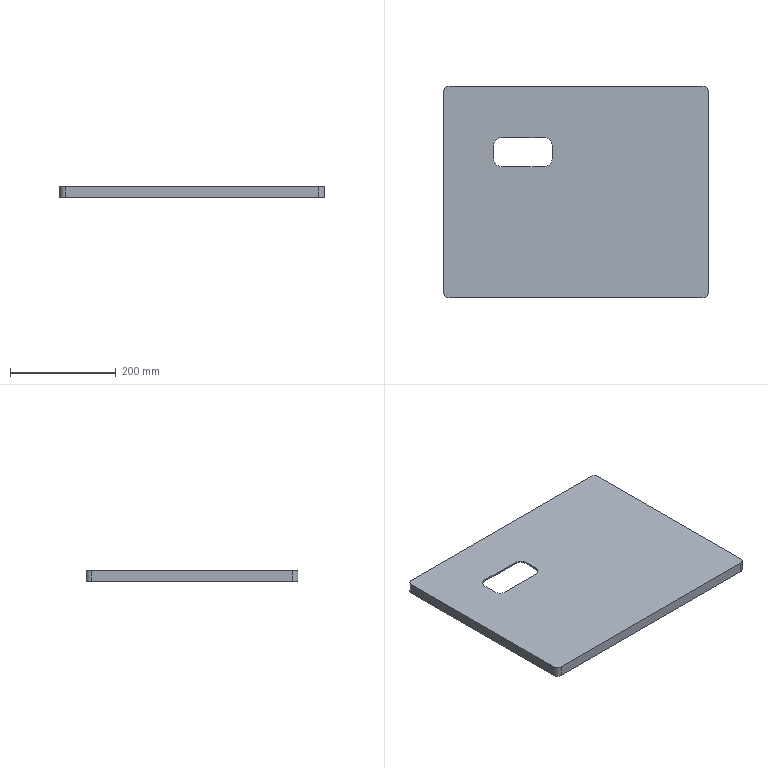Component | SolidWorks | LX-TSJ-16-1 | 1 solid | 27 faces | box 500 x 400 x 20 mm | volume 672509 mm3 | plane 15 | cylinder 12 | commonest cylinder face diameters 20 x4 14 x4 30 x4
STEP:
#1=COLOUR_RGB('',0.7922,0.8196,0.9333);
#2=FILL_AREA_STYLE_COLOUR('',#1);
#3=FILL_AREA_STYLE('',(#2));
#4=SURFACE_STYLE_FILL_AREA(#3);
#5=SURFACE_SIDE_STYLE('',(#4));
#6=SURFACE_STYLE_USAGE(.BOTH.,#5);
#7=PRESENTATION_STYLE_ASSIGNMENT((#6));
#8=CARTESIAN_POINT('',(-7.413,-19.336,-5.681));
#9=VERTEX_POINT('',#8);
#10=CARTESIAN_POINT('',(-7.413,-20.326,-5.681));
#11=VERTEX_POINT('',#10);
#12=CARTESIAN_POINT('',(-7.413,-30.275,-5.681));
#13=DIRECTION('',(0.,-1.,-0.));
#14=VECTOR('',#13,39.37);
#15=LINE('',#12,#14);
#16=EDGE_CURVE('',#9,#11,#15,.T.);
#17=ORIENTED_EDGE('',*,*,#16,.T.);
#18=CARTESIAN_POINT('',(-8.004,-20.917,-5.681));
#19=VERTEX_POINT('',#18);
#20=CARTESIAN_POINT('',(-8.004,-20.326,-5.681));
#21=DIRECTION('',(0.,0.,-1.));
#22=DIRECTION('',(-1.,0.,0.));
#23=AXIS2_PLACEMENT_3D('',#20,#21,#22);
#24=CIRCLE('',#23,0.5906);
#25=EDGE_CURVE('',#11,#19,#24,.T.);
#26=ORIENTED_EDGE('',*,*,#25,.T.);
#27=CARTESIAN_POINT('',(-11.166,-20.917,-5.681));
#28=VERTEX_POINT('',#27);
#29=CARTESIAN_POINT('',(3.818,-20.917,-5.681));
#30=DIRECTION('',(-1.,-0.,-0.));
#31=VECTOR('',#30,39.37);
#32=LINE('',#29,#31);
#33=EDGE_CURVE('',#19,#28,#32,.T.);
#34=ORIENTED_EDGE('',*,*,#33,.T.);
#35=CARTESIAN_POINT('',(-11.756,-20.326,-5.681));
#36=VERTEX_POINT('',#35);
#37=CARTESIAN_POINT('',(-11.166,-20.326,-5.681));
#38=DIRECTION('',(0.,0.,-1.));
#39=DIRECTION('',(-1.,0.,0.));
#40=AXIS2_PLACEMENT_3D('',#37,#38,#39);
#41=CIRCLE('',#40,0.5906);
#42=EDGE_CURVE('',#28,#36,#41,.T.);
#43=ORIENTED_EDGE('',*,*,#42,.T.);
#44=CARTESIAN_POINT('',(-11.756,-19.336,-5.681));
#45=VERTEX_POINT('',#44);
#46=CARTESIAN_POINT('',(-11.756,-30.275,-5.681));
#47=DIRECTION('',(-0.,1.,0.));
#48=VECTOR('',#47,39.37);
#49=LINE('',#46,#48);
#50=EDGE_CURVE('',#36,#45,#49,.T.);
#51=ORIENTED_EDGE('',*,*,#50,.T.);
#52=CARTESIAN_POINT('',(-11.166,-18.745,-5.681));
#53=VERTEX_POINT('',#52);
#54=CARTESIAN_POINT('',(-11.166,-19.336,-5.681));
#55=DIRECTION('',(0.,0.,-1.));
#56=DIRECTION('',(-1.,0.,0.));
#57=AXIS2_PLACEMENT_3D('',#54,#55,#56);
#58=CIRCLE('',#57,0.5906);
#59=EDGE_CURVE('',#45,#53,#58,.T.);
#60=ORIENTED_EDGE('',*,*,#59,.T.);
#61=CARTESIAN_POINT('',(-8.004,-18.745,-5.681));
#62=VERTEX_POINT('',#61);
#63=CARTESIAN_POINT('',(3.818,-18.745,-5.681));
#64=DIRECTION('',(1.,0.,0.));
#65=VECTOR('',#64,39.37);
#66=LINE('',#63,#65);
#67=EDGE_CURVE('',#53,#62,#66,.T.);
#68=ORIENTED_EDGE('',*,*,#67,.T.);
#69=CARTESIAN_POINT('',(-8.004,-19.336,-5.681));
#70=DIRECTION('',(0.,0.,-1.));
#71=DIRECTION('',(-1.,0.,0.));
#72=AXIS2_PLACEMENT_3D('',#69,#70,#71);
#73=CIRCLE('',#72,0.5906);
#74=EDGE_CURVE('',#62,#9,#73,.T.);
#75=ORIENTED_EDGE('',*,*,#74,.T.);
#76=EDGE_LOOP('',(#17,#26,#34,#43,#51,#60,#68,#75));
#77=FACE_BOUND('',#76,.T.);
#78=CARTESIAN_POINT('',(4.212,-15.314,-5.681));
#79=VERTEX_POINT('',#78);
#80=CARTESIAN_POINT('',(4.212,-30.275,-5.681));
#81=VERTEX_POINT('',#80);
#82=CARTESIAN_POINT('',(4.212,-30.275,-5.681));
#83=DIRECTION('',(0.,-1.,-0.));
#84=VECTOR('',#83,39.37);
#85=LINE('',#82,#84);
#86=EDGE_CURVE('',#79,#81,#85,.T.);
#87=ORIENTED_EDGE('',*,*,#86,.F.);
#88=CARTESIAN_POINT('',(3.818,-14.92,-5.681));
#89=VERTEX_POINT('',#88);
#90=CARTESIAN_POINT('',(3.818,-15.314,-5.681));
#91=DIRECTION('',(0.,0.,-1.));
#92=DIRECTION('',(1.,0.,0.));
#93=AXIS2_PLACEMENT_3D('',#90,#91,#92);
#94=CIRCLE('',#93,0.3937);
#95=EDGE_CURVE('',#89,#79,#94,.T.);
#96=ORIENTED_EDGE('',*,*,#95,.F.);
#97=CARTESIAN_POINT('',(-15.08,-14.92,-5.681));
#98=VERTEX_POINT('',#97);
#99=CARTESIAN_POINT('',(3.818,-14.92,-5.681));
#100=DIRECTION('',(1.,0.,0.));
#101=VECTOR('',#100,39.37);
#102=LINE('',#99,#101);
#103=EDGE_CURVE('',#98,#89,#102,.T.);
#104=ORIENTED_EDGE('',*,*,#103,.F.);
#105=CARTESIAN_POINT('',(-15.473,-15.314,-5.681));
#106=VERTEX_POINT('',#105);
#107=CARTESIAN_POINT('',(-15.08,-15.314,-5.681));
#108=DIRECTION('',(0.,0.,-1.));
#109=DIRECTION('',(1.,0.,0.));
#110=AXIS2_PLACEMENT_3D('',#107,#108,#109);
#111=CIRCLE('',#110,0.3937);
#112=EDGE_CURVE('',#106,#98,#111,.T.);
#113=ORIENTED_EDGE('',*,*,#112,.F.);
#114=CARTESIAN_POINT('',(-15.473,-30.275,-5.681));
#115=VERTEX_POINT('',#114);
#116=CARTESIAN_POINT('',(-15.473,-30.275,-5.681));
#117=DIRECTION('',(-0.,1.,0.));
#118=VECTOR('',#117,39.37);
#119=LINE('',#116,#118);
#120=EDGE_CURVE('',#115,#106,#119,.T.);
#121=ORIENTED_EDGE('',*,*,#120,.F.);
#122=CARTESIAN_POINT('',(-15.08,-30.668,-5.681));
#123=VERTEX_POINT('',#122);
#124=CARTESIAN_POINT('',(-15.08,-30.275,-5.681));
#125=DIRECTION('',(0.,0.,-1.));
#126=DIRECTION('',(1.,0.,0.));
#127=AXIS2_PLACEMENT_3D('',#124,#125,#126);
#128=CIRCLE('',#127,0.3937);
#129=EDGE_CURVE('',#123,#115,#128,.T.);
#130=ORIENTED_EDGE('',*,*,#129,.F.);
#131=CARTESIAN_POINT('',(3.818,-30.668,-5.681));
#132=VERTEX_POINT('',#131);
#133=CARTESIAN_POINT('',(3.818,-30.668,-5.681));
#134=DIRECTION('',(-1.,-0.,-0.));
#135=VECTOR('',#134,39.37);
#136=LINE('',#133,#135);
#137=EDGE_CURVE('',#132,#123,#136,.T.);
#138=ORIENTED_EDGE('',*,*,#137,.F.);
#139=CARTESIAN_POINT('',(3.818,-30.275,-5.681));
#140=DIRECTION('',(0.,0.,-1.));
#141=DIRECTION('',(1.,0.,0.));
#142=AXIS2_PLACEMENT_3D('',#139,#140,#141);
#143=CIRCLE('',#142,0.3937);
#144=EDGE_CURVE('',#81,#132,#143,.T.);
#145=ORIENTED_EDGE('',*,*,#144,.F.);
#146=EDGE_LOOP('',(#87,#96,#104,#113,#121,#130,#138,#145));
#147=FACE_OUTER_BOUND('',#146,.T.);
#148=CARTESIAN_POINT('',(3.818,-30.275,-5.681));
#149=DIRECTION('',(0.,0.,-1.));
#150=DIRECTION('',(-1.,-0.,-0.));
#151=AXIS2_PLACEMENT_3D('',#148,#149,#150);
#152=PLANE('',#151);
#153=ADVANCED_FACE('',(#77,#147),#152,.F.);
#154=CARTESIAN_POINT('',(3.818,-30.668,-6.468));
#155=VERTEX_POINT('',#154);
#156=CARTESIAN_POINT('',(4.212,-30.275,-6.468));
#157=VERTEX_POINT('',#156);
#158=CARTESIAN_POINT('',(3.818,-30.275,-6.468));
#159=DIRECTION('',(-0.,-0.,1.));
#160=DIRECTION('',(1.,0.,0.));
#161=AXIS2_PLACEMENT_3D('',#158,#159,#160);
#162=CIRCLE('',#161,0.3937);
#163=EDGE_CURVE('',#155,#157,#162,.T.);
#164=ORIENTED_EDGE('',*,*,#163,.T.);
#165=CARTESIAN_POINT('',(4.212,-30.275,-6.468));
#166=DIRECTION('',(-0.,-0.,1.));
#167=VECTOR('',#166,39.37);
#168=LINE('',#165,#167);
#169=EDGE_CURVE('',#157,#81,#168,.T.);
#170=ORIENTED_EDGE('',*,*,#169,.T.);
#171=ORIENTED_EDGE('',*,*,#144,.T.);
#172=CARTESIAN_POINT('',(3.818,-30.668,-6.468));
#173=DIRECTION('',(0.,0.,-1.));
#174=VECTOR('',#173,39.37);
#175=LINE('',#172,#174);
#176=EDGE_CURVE('',#132,#155,#175,.T.);
#177=ORIENTED_EDGE('',*,*,#176,.T.);
#178=EDGE_LOOP('',(#164,#170,#171,#177));
#179=FACE_OUTER_BOUND('',#178,.T.);
#180=CARTESIAN_POINT('',(3.818,-30.275,-6.468));
#181=DIRECTION('',(-0.,-0.,1.));
#182=DIRECTION('',(1.,0.,0.));
#183=AXIS2_PLACEMENT_3D('',#180,#181,#182);
#184=CYLINDRICAL_SURFACE('',#183,0.3937);
#185=ADVANCED_FACE('',(#179),#184,.T.);
#186=ORIENTED_EDGE('',*,*,#169,.F.);
#187=CARTESIAN_POINT('',(4.212,-15.314,-6.468));
#188=VERTEX_POINT('',#187);
#189=CARTESIAN_POINT('',(4.212,-15.314,-6.468));
#190=DIRECTION('',(0.,-1.,-0.));
#191=VECTOR('',#190,39.37);
#192=LINE('',#189,#191);
#193=EDGE_CURVE('',#188,#157,#192,.T.);
#194=ORIENTED_EDGE('',*,*,#193,.F.);
#195=CARTESIAN_POINT('',(4.212,-15.314,-6.468));
#196=DIRECTION('',(0.,0.,-1.));
#197=VECTOR('',#196,39.37);
#198=LINE('',#195,#197);
#199=EDGE_CURVE('',#79,#188,#198,.T.);
#200=ORIENTED_EDGE('',*,*,#199,.F.);
#201=ORIENTED_EDGE('',*,*,#86,.T.);
#202=EDGE_LOOP('',(#186,#194,#200,#201));
#203=FACE_OUTER_BOUND('',#202,.T.);
#204=CARTESIAN_POINT('',(4.212,-15.314,-6.468));
#205=DIRECTION('',(-1.,-0.,-0.));
#206=DIRECTION('',(-0.,1.,0.));
#207=AXIS2_PLACEMENT_3D('',#204,#205,#206);
#208=PLANE('',#207);
#209=ADVANCED_FACE('',(#203),#208,.F.);
#210=CARTESIAN_POINT('',(3.818,-14.92,-6.468));
#211=VERTEX_POINT('',#210);
#212=CARTESIAN_POINT('',(3.818,-15.314,-6.468));
#213=DIRECTION('',(-0.,-0.,1.));
#214=DIRECTION('',(1.,0.,0.));
#215=AXIS2_PLACEMENT_3D('',#212,#213,#214);
#216=CIRCLE('',#215,0.3937);
#217=EDGE_CURVE('',#188,#211,#216,.T.);
#218=ORIENTED_EDGE('',*,*,#217,.T.);
#219=CARTESIAN_POINT('',(3.818,-14.92,-6.468));
#220=DIRECTION('',(-0.,-0.,1.));
#221=VECTOR('',#220,39.37);
#222=LINE('',#219,#221);
#223=EDGE_CURVE('',#211,#89,#222,.T.);
#224=ORIENTED_EDGE('',*,*,#223,.T.);
#225=ORIENTED_EDGE('',*,*,#95,.T.);
#226=ORIENTED_EDGE('',*,*,#199,.T.);
#227=EDGE_LOOP('',(#218,#224,#225,#226));
#228=FACE_OUTER_BOUND('',#227,.T.);
#229=CARTESIAN_POINT('',(3.818,-15.314,-6.468));
#230=DIRECTION('',(-0.,-0.,1.));
#231=DIRECTION('',(1.,0.,0.));
#232=AXIS2_PLACEMENT_3D('',#229,#230,#231);
#233=CYLINDRICAL_SURFACE('',#232,0.3937);
#234=ADVANCED_FACE('',(#228),#233,.T.);
#235=ORIENTED_EDGE('',*,*,#223,.F.);
#236=CARTESIAN_POINT('',(-15.08,-14.92,-6.468));
#237=VERTEX_POINT('',#236);
#238=CARTESIAN_POINT('',(3.818,-14.92,-6.468));
#239=DIRECTION('',(1.,0.,0.));
#240=VECTOR('',#239,39.37);
#241=LINE('',#238,#240);
#242=EDGE_CURVE('',#237,#211,#241,.T.);
#243=ORIENTED_EDGE('',*,*,#242,.F.);
#244=CARTESIAN_POINT('',(-15.08,-14.92,-6.468));
#245=DIRECTION('',(0.,0.,-1.));
#246=VECTOR('',#245,39.37);
#247=LINE('',#244,#246);
#248=EDGE_CURVE('',#98,#237,#247,.T.);
#249=ORIENTED_EDGE('',*,*,#248,.F.);
#250=ORIENTED_EDGE('',*,*,#103,.T.);
#251=EDGE_LOOP('',(#235,#243,#249,#250));
#252=FACE_OUTER_BOUND('',#251,.T.);
#253=CARTESIAN_POINT('',(3.818,-14.92,-6.468));
#254=DIRECTION('',(0.,-1.,-0.));
#255=DIRECTION('',(-0.,-0.,1.));
#256=AXIS2_PLACEMENT_3D('',#253,#254,#255);
#257=PLANE('',#256);
#258=ADVANCED_FACE('',(#252),#257,.F.);
#259=CARTESIAN_POINT('',(-15.473,-15.314,-6.468));
#260=VERTEX_POINT('',#259);
#261=CARTESIAN_POINT('',(-15.08,-15.314,-6.468));
#262=DIRECTION('',(-0.,-0.,1.));
#263=DIRECTION('',(1.,0.,0.));
#264=AXIS2_PLACEMENT_3D('',#261,#262,#263);
#265=CIRCLE('',#264,0.3937);
#266=EDGE_CURVE('',#237,#260,#265,.T.);
#267=ORIENTED_EDGE('',*,*,#266,.T.);
#268=CARTESIAN_POINT('',(-15.473,-15.314,-6.468));
#269=DIRECTION('',(-0.,-0.,1.));
#270=VECTOR('',#269,39.37);
#271=LINE('',#268,#270);
#272=EDGE_CURVE('',#260,#106,#271,.T.);
#273=ORIENTED_EDGE('',*,*,#272,.T.);
#274=ORIENTED_EDGE('',*,*,#112,.T.);
#275=ORIENTED_EDGE('',*,*,#248,.T.);
#276=EDGE_LOOP('',(#267,#273,#274,#275));
#277=FACE_OUTER_BOUND('',#276,.T.);
#278=CARTESIAN_POINT('',(-15.08,-15.314,-6.468));
#279=DIRECTION('',(-0.,-0.,1.));
#280=DIRECTION('',(1.,0.,0.));
#281=AXIS2_PLACEMENT_3D('',#278,#279,#280);
#282=CYLINDRICAL_SURFACE('',#281,0.3937);
#283=ADVANCED_FACE('',(#277),#282,.T.);
#284=ORIENTED_EDGE('',*,*,#272,.F.);
#285=CARTESIAN_POINT('',(-15.473,-30.275,-6.468));
#286=VERTEX_POINT('',#285);
#287=CARTESIAN_POINT('',(-15.473,-15.314,-6.468));
#288=DIRECTION('',(-0.,1.,0.));
#289=VECTOR('',#288,39.37);
#290=LINE('',#287,#289);
#291=EDGE_CURVE('',#286,#260,#290,.T.);
#292=ORIENTED_EDGE('',*,*,#291,.F.);
#293=CARTESIAN_POINT('',(-15.473,-30.275,-6.468));
#294=DIRECTION('',(0.,0.,-1.));
#295=VECTOR('',#294,39.37);
#296=LINE('',#293,#295);
#297=EDGE_CURVE('',#115,#286,#296,.T.);
#298=ORIENTED_EDGE('',*,*,#297,.F.);
#299=ORIENTED_EDGE('',*,*,#120,.T.);
#300=EDGE_LOOP('',(#284,#292,#298,#299));
#301=FACE_OUTER_BOUND('',#300,.T.);
#302=CARTESIAN_POINT('',(-15.473,-15.314,-6.468));
#303=DIRECTION('',(1.,0.,0.));
#304=DIRECTION('',(0.,-1.,-0.));
#305=AXIS2_PLACEMENT_3D('',#302,#303,#304);
#306=PLANE('',#305);
#307=ADVANCED_FACE('',(#301),#306,.F.);
#308=CARTESIAN_POINT('',(-15.08,-30.668,-6.468));
#309=VERTEX_POINT('',#308);
#310=CARTESIAN_POINT('',(-15.08,-30.275,-6.468));
#311=DIRECTION('',(-0.,-0.,1.));
#312=DIRECTION('',(1.,0.,0.));
#313=AXIS2_PLACEMENT_3D('',#310,#311,#312);
#314=CIRCLE('',#313,0.3937);
#315=EDGE_CURVE('',#286,#309,#314,.T.);
#316=ORIENTED_EDGE('',*,*,#315,.T.);
#317=CARTESIAN_POINT('',(-15.08,-30.668,-6.468));
#318=DIRECTION('',(-0.,-0.,1.));
#319=VECTOR('',#318,39.37);
#320=LINE('',#317,#319);
#321=EDGE_CURVE('',#309,#123,#320,.T.);
#322=ORIENTED_EDGE('',*,*,#321,.T.);
#323=ORIENTED_EDGE('',*,*,#129,.T.);
#324=ORIENTED_EDGE('',*,*,#297,.T.);
#325=EDGE_LOOP('',(#316,#322,#323,#324));
#326=FACE_OUTER_BOUND('',#325,.T.);
#327=CARTESIAN_POINT('',(-15.08,-30.275,-6.468));
#328=DIRECTION('',(-0.,-0.,1.));
#329=DIRECTION('',(1.,0.,0.));
#330=AXIS2_PLACEMENT_3D('',#327,#328,#329);
#331=CYLINDRICAL_SURFACE('',#330,0.3937);
#332=ADVANCED_FACE('',(#326),#331,.T.);
#333=ORIENTED_EDGE('',*,*,#321,.F.);
#334=CARTESIAN_POINT('',(3.818,-30.668,-6.468));
#335=DIRECTION('',(-1.,-0.,-0.));
#336=VECTOR('',#335,39.37);
#337=LINE('',#334,#336);
#338=EDGE_CURVE('',#155,#309,#337,.T.);
#339=ORIENTED_EDGE('',*,*,#338,.F.);
#340=ORIENTED_EDGE('',*,*,#176,.F.);
#341=ORIENTED_EDGE('',*,*,#137,.T.);
#342=EDGE_LOOP('',(#333,#339,#340,#341));
#343=FACE_OUTER_BOUND('',#342,.T.);
#344=CARTESIAN_POINT('',(3.818,-30.668,-6.468));
#345=DIRECTION('',(-0.,1.,0.));
#346=DIRECTION('',(0.,0.,-1.));
#347=AXIS2_PLACEMENT_3D('',#344,#345,#346);
#348=PLANE('',#347);
#349=ADVANCED_FACE('',(#343),#348,.F.);
#350=ORIENTED_EDGE('',*,*,#217,.F.);
#351=ORIENTED_EDGE('',*,*,#193,.T.);
#352=ORIENTED_EDGE('',*,*,#163,.F.);
#353=ORIENTED_EDGE('',*,*,#338,.T.);
#354=ORIENTED_EDGE('',*,*,#315,.F.);
#355=ORIENTED_EDGE('',*,*,#291,.T.);
#356=ORIENTED_EDGE('',*,*,#266,.F.);
#357=ORIENTED_EDGE('',*,*,#242,.T.);
#358=EDGE_LOOP('',(#350,#351,#352,#353,#354,#355,#356,#357));
#359=FACE_OUTER_BOUND('',#358,.T.);
#360=CARTESIAN_POINT('',(-15.355,-30.275,-6.468));
#361=VERTEX_POINT('',#360);
#362=CARTESIAN_POINT('',(-15.08,-30.55,-6.468));
#363=VERTEX_POINT('',#362);
#364=CARTESIAN_POINT('',(-15.08,-30.275,-6.468));
#365=DIRECTION('',(-0.,-0.,1.));
#366=DIRECTION('',(1.,0.,0.));
#367=AXIS2_PLACEMENT_3D('',#364,#365,#366);
#368=CIRCLE('',#367,0.2756);
#369=EDGE_CURVE('',#361,#363,#368,.T.);
#370=ORIENTED_EDGE('',*,*,#369,.T.);
#371=CARTESIAN_POINT('',(3.818,-30.55,-6.468));
#372=VERTEX_POINT('',#371);
#373=CARTESIAN_POINT('',(3.818,-30.55,-6.468));
#374=DIRECTION('',(1.,0.,0.));
#375=VECTOR('',#374,39.37);
#376=LINE('',#373,#375);
#377=EDGE_CURVE('',#363,#372,#376,.T.);
#378=ORIENTED_EDGE('',*,*,#377,.T.);
#379=CARTESIAN_POINT('',(4.094,-30.275,-6.468));
#380=VERTEX_POINT('',#379);
#381=CARTESIAN_POINT('',(3.818,-30.275,-6.468));
#382=DIRECTION('',(-0.,-0.,1.));
#383=DIRECTION('',(1.,0.,0.));
#384=AXIS2_PLACEMENT_3D('',#381,#382,#383);
#385=CIRCLE('',#384,0.2756);
#386=EDGE_CURVE('',#372,#380,#385,.T.);
#387=ORIENTED_EDGE('',*,*,#386,.T.);
#388=CARTESIAN_POINT('',(4.094,-15.314,-6.468));
#389=VERTEX_POINT('',#388);
#390=CARTESIAN_POINT('',(4.094,-30.275,-6.468));
#391=DIRECTION('',(-0.,1.,0.));
#392=VECTOR('',#391,39.37);
#393=LINE('',#390,#392);
#394=EDGE_CURVE('',#380,#389,#393,.T.);
#395=ORIENTED_EDGE('',*,*,#394,.T.);
#396=CARTESIAN_POINT('',(3.818,-15.038,-6.468));
#397=VERTEX_POINT('',#396);
#398=CARTESIAN_POINT('',(3.818,-15.314,-6.468));
#399=DIRECTION('',(-0.,-0.,1.));
#400=DIRECTION('',(1.,0.,0.));
#401=AXIS2_PLACEMENT_3D('',#398,#399,#400);
#402=CIRCLE('',#401,0.2756);
#403=EDGE_CURVE('',#389,#397,#402,.T.);
#404=ORIENTED_EDGE('',*,*,#403,.T.);
#405=CARTESIAN_POINT('',(-15.08,-15.038,-6.468));
#406=VERTEX_POINT('',#405);
#407=CARTESIAN_POINT('',(3.818,-15.038,-6.468));
#408=DIRECTION('',(-1.,-0.,-0.));
#409=VECTOR('',#408,39.37);
#410=LINE('',#407,#409);
#411=EDGE_CURVE('',#397,#406,#410,.T.);
#412=ORIENTED_EDGE('',*,*,#411,.T.);
#413=CARTESIAN_POINT('',(-15.355,-15.314,-6.468));
#414=VERTEX_POINT('',#413);
#415=CARTESIAN_POINT('',(-15.08,-15.314,-6.468));
#416=DIRECTION('',(-0.,-0.,1.));
#417=DIRECTION('',(1.,0.,0.));
#418=AXIS2_PLACEMENT_3D('',#415,#416,#417);
#419=CIRCLE('',#418,0.2756);
#420=EDGE_CURVE('',#406,#414,#419,.T.);
#421=ORIENTED_EDGE('',*,*,#420,.T.);
#422=CARTESIAN_POINT('',(-15.355,-30.275,-6.468));
#423=DIRECTION('',(0.,-1.,-0.));
#424=VECTOR('',#423,39.37);
#425=LINE('',#422,#424);
#426=EDGE_CURVE('',#414,#361,#425,.T.);
#427=ORIENTED_EDGE('',*,*,#426,.T.);
#428=EDGE_LOOP('',(#370,#378,#387,#395,#404,#412,#421,#427));
#429=FACE_BOUND('',#428,.T.);
#430=CARTESIAN_POINT('',(3.818,-30.275,-6.468));
#431=DIRECTION('',(0.,0.,-1.));
#432=DIRECTION('',(-1.,-0.,-0.));
#433=AXIS2_PLACEMENT_3D('',#430,#431,#432);
#434=PLANE('',#433);
#435=ADVANCED_FACE('',(#359,#429),#434,.T.);
#436=ORIENTED_EDGE('',*,*,#377,.F.);
#437=CARTESIAN_POINT('',(-15.08,-30.55,-5.799));
#438=VERTEX_POINT('',#437);
#439=CARTESIAN_POINT('',(-15.08,-30.55,-6.468));
#440=DIRECTION('',(-0.,-0.,1.));
#441=VECTOR('',#440,39.37);
#442=LINE('',#439,#441);
#443=EDGE_CURVE('',#363,#438,#442,.T.);
#444=ORIENTED_EDGE('',*,*,#443,.T.);
#445=CARTESIAN_POINT('',(3.818,-30.55,-5.799));
#446=VERTEX_POINT('',#445);
#447=CARTESIAN_POINT('',(3.818,-30.55,-5.799));
#448=DIRECTION('',(1.,0.,0.));
#449=VECTOR('',#448,39.37);
#450=LINE('',#447,#449);
#451=EDGE_CURVE('',#438,#446,#450,.T.);
#452=ORIENTED_EDGE('',*,*,#451,.T.);
#453=CARTESIAN_POINT('',(3.818,-30.55,-6.468));
#454=DIRECTION('',(0.,0.,-1.));
#455=VECTOR('',#454,39.37);
#456=LINE('',#453,#455);
#457=EDGE_CURVE('',#446,#372,#456,.T.);
#458=ORIENTED_EDGE('',*,*,#457,.T.);
#459=EDGE_LOOP('',(#436,#444,#452,#458));
#460=FACE_OUTER_BOUND('',#459,.T.);
#461=CARTESIAN_POINT('',(3.818,-30.55,-6.468));
#462=DIRECTION('',(-0.,1.,0.));
#463=DIRECTION('',(0.,0.,-1.));
#464=AXIS2_PLACEMENT_3D('',#461,#462,#463);
#465=PLANE('',#464);
#466=ADVANCED_FACE('',(#460),#465,.T.);
#467=ORIENTED_EDGE('',*,*,#443,.F.);
#468=ORIENTED_EDGE('',*,*,#369,.F.);
#469=CARTESIAN_POINT('',(-15.355,-30.275,-5.799));
#470=VERTEX_POINT('',#469);
#471=CARTESIAN_POINT('',(-15.355,-30.275,-6.468));
#472=DIRECTION('',(0.,0.,-1.));
#473=VECTOR('',#472,39.37);
#474=LINE('',#471,#473);
#475=EDGE_CURVE('',#470,#361,#474,.T.);
#476=ORIENTED_EDGE('',*,*,#475,.F.);
#477=CARTESIAN_POINT('',(-15.08,-30.275,-5.799));
#478=DIRECTION('',(0.,0.,-1.));
#479=DIRECTION('',(1.,0.,0.));
#480=AXIS2_PLACEMENT_3D('',#477,#478,#479);
#481=CIRCLE('',#480,0.2756);
#482=EDGE_CURVE('',#438,#470,#481,.T.);
#483=ORIENTED_EDGE('',*,*,#482,.F.);
#484=EDGE_LOOP('',(#467,#468,#476,#483));
#485=FACE_OUTER_BOUND('',#484,.T.);
#486=CARTESIAN_POINT('',(-15.08,-30.275,-6.468));
#487=DIRECTION('',(-0.,-0.,1.));
#488=DIRECTION('',(1.,0.,0.));
#489=AXIS2_PLACEMENT_3D('',#486,#487,#488);
#490=CYLINDRICAL_SURFACE('',#489,0.2756);
#491=ADVANCED_FACE('',(#485),#490,.F.);
#492=ORIENTED_EDGE('',*,*,#426,.F.);
#493=CARTESIAN_POINT('',(-15.355,-15.314,-5.799));
#494=VERTEX_POINT('',#493);
#495=CARTESIAN_POINT('',(-15.355,-15.314,-6.468));
#496=DIRECTION('',(-0.,-0.,1.));
#497=VECTOR('',#496,39.37);
#498=LINE('',#495,#497);
#499=EDGE_CURVE('',#414,#494,#498,.T.);
#500=ORIENTED_EDGE('',*,*,#499,.T.);
#501=CARTESIAN_POINT('',(-15.355,-15.314,-5.799));
#502=DIRECTION('',(0.,-1.,-0.));
#503=VECTOR('',#502,39.37);
#504=LINE('',#501,#503);
#505=EDGE_CURVE('',#494,#470,#504,.T.);
#506=ORIENTED_EDGE('',*,*,#505,.T.);
#507=ORIENTED_EDGE('',*,*,#475,.T.);
#508=EDGE_LOOP('',(#492,#500,#506,#507));
#509=FACE_OUTER_BOUND('',#508,.T.);
#510=CARTESIAN_POINT('',(-15.355,-15.314,-6.468));
#511=DIRECTION('',(1.,0.,0.));
#512=DIRECTION('',(0.,-1.,-0.));
#513=AXIS2_PLACEMENT_3D('',#510,#511,#512);
#514=PLANE('',#513);
#515=ADVANCED_FACE('',(#509),#514,.T.);
#516=ORIENTED_EDGE('',*,*,#499,.F.);
#517=ORIENTED_EDGE('',*,*,#420,.F.);
#518=CARTESIAN_POINT('',(-15.08,-15.038,-5.799));
#519=VERTEX_POINT('',#518);
#520=CARTESIAN_POINT('',(-15.08,-15.038,-6.468));
#521=DIRECTION('',(0.,0.,-1.));
#522=VECTOR('',#521,39.37);
#523=LINE('',#520,#522);
#524=EDGE_CURVE('',#519,#406,#523,.T.);
#525=ORIENTED_EDGE('',*,*,#524,.F.);
#526=CARTESIAN_POINT('',(-15.08,-15.314,-5.799));
#527=DIRECTION('',(0.,0.,-1.));
#528=DIRECTION('',(1.,0.,0.));
#529=AXIS2_PLACEMENT_3D('',#526,#527,#528);
#530=CIRCLE('',#529,0.2756);
#531=EDGE_CURVE('',#494,#519,#530,.T.);
#532=ORIENTED_EDGE('',*,*,#531,.F.);
#533=EDGE_LOOP('',(#516,#517,#525,#532));
#534=FACE_OUTER_BOUND('',#533,.T.);
#535=CARTESIAN_POINT('',(-15.08,-15.314,-6.468));
#536=DIRECTION('',(-0.,-0.,1.));
#537=DIRECTION('',(1.,0.,0.));
#538=AXIS2_PLACEMENT_3D('',#535,#536,#537);
#539=CYLINDRICAL_SURFACE('',#538,0.2756);
#540=ADVANCED_FACE('',(#534),#539,.F.);
#541=ORIENTED_EDGE('',*,*,#411,.F.);
#542=CARTESIAN_POINT('',(3.818,-15.038,-5.799));
#543=VERTEX_POINT('',#542);
#544=CARTESIAN_POINT('',(3.818,-15.038,-6.468));
#545=DIRECTION('',(-0.,-0.,1.));
#546=VECTOR('',#545,39.37);
#547=LINE('',#544,#546);
#548=EDGE_CURVE('',#397,#543,#547,.T.);
#549=ORIENTED_EDGE('',*,*,#548,.T.);
#550=CARTESIAN_POINT('',(3.818,-15.038,-5.799));
#551=DIRECTION('',(-1.,-0.,-0.));
#552=VECTOR('',#551,39.37);
#553=LINE('',#550,#552);
#554=EDGE_CURVE('',#543,#519,#553,.T.);
#555=ORIENTED_EDGE('',*,*,#554,.T.);
#556=ORIENTED_EDGE('',*,*,#524,.T.);
#557=EDGE_LOOP('',(#541,#549,#555,#556));
#558=FACE_OUTER_BOUND('',#557,.T.);
#559=CARTESIAN_POINT('',(3.818,-15.038,-6.468));
#560=DIRECTION('',(0.,-1.,-0.));
#561=DIRECTION('',(-0.,-0.,1.));
#562=AXIS2_PLACEMENT_3D('',#559,#560,#561);
#563=PLANE('',#562);
#564=ADVANCED_FACE('',(#558),#563,.T.);
#565=ORIENTED_EDGE('',*,*,#548,.F.);
#566=ORIENTED_EDGE('',*,*,#403,.F.);
#567=CARTESIAN_POINT('',(4.094,-15.314,-5.799));
#568=VERTEX_POINT('',#567);
#569=CARTESIAN_POINT('',(4.094,-15.314,-6.468));
#570=DIRECTION('',(0.,0.,-1.));
#571=VECTOR('',#570,39.37);
#572=LINE('',#569,#571);
#573=EDGE_CURVE('',#568,#389,#572,.T.);
#574=ORIENTED_EDGE('',*,*,#573,.F.);
#575=CARTESIAN_POINT('',(3.818,-15.314,-5.799));
#576=DIRECTION('',(0.,0.,-1.));
#577=DIRECTION('',(1.,0.,0.));
#578=AXIS2_PLACEMENT_3D('',#575,#576,#577);
#579=CIRCLE('',#578,0.2756);
#580=EDGE_CURVE('',#543,#568,#579,.T.);
#581=ORIENTED_EDGE('',*,*,#580,.F.);
#582=EDGE_LOOP('',(#565,#566,#574,#581));
#583=FACE_OUTER_BOUND('',#582,.T.);
#584=CARTESIAN_POINT('',(3.818,-15.314,-6.468));
#585=DIRECTION('',(-0.,-0.,1.));
#586=DIRECTION('',(1.,0.,0.));
#587=AXIS2_PLACEMENT_3D('',#584,#585,#586);
#588=CYLINDRICAL_SURFACE('',#587,0.2756);
#589=ADVANCED_FACE('',(#583),#588,.F.);
#590=ORIENTED_EDGE('',*,*,#394,.F.);
#591=CARTESIAN_POINT('',(4.094,-30.275,-5.799));
#592=VERTEX_POINT('',#591);
#593=CARTESIAN_POINT('',(4.094,-30.275,-6.468));
#594=DIRECTION('',(-0.,-0.,1.));
#595=VECTOR('',#594,39.37);
#596=LINE('',#593,#595);
#597=EDGE_CURVE('',#380,#592,#596,.T.);
#598=ORIENTED_EDGE('',*,*,#597,.T.);
#599=CARTESIAN_POINT('',(4.094,-15.314,-5.799));
#600=DIRECTION('',(-0.,1.,0.));
#601=VECTOR('',#600,39.37);
#602=LINE('',#599,#601);
#603=EDGE_CURVE('',#592,#568,#602,.T.);
#604=ORIENTED_EDGE('',*,*,#603,.T.);
#605=ORIENTED_EDGE('',*,*,#573,.T.);
#606=EDGE_LOOP('',(#590,#598,#604,#605));
#607=FACE_OUTER_BOUND('',#606,.T.);
#608=CARTESIAN_POINT('',(4.094,-15.314,-6.468));
#609=DIRECTION('',(-1.,-0.,-0.));
#610=DIRECTION('',(-0.,1.,0.));
#611=AXIS2_PLACEMENT_3D('',#608,#609,#610);
#612=PLANE('',#611);
#613=ADVANCED_FACE('',(#607),#612,.T.);
#614=ORIENTED_EDGE('',*,*,#597,.F.);
#615=ORIENTED_EDGE('',*,*,#386,.F.);
#616=ORIENTED_EDGE('',*,*,#457,.F.);
#617=CARTESIAN_POINT('',(3.818,-30.275,-5.799));
#618=DIRECTION('',(0.,0.,-1.));
#619=DIRECTION('',(1.,0.,0.));
#620=AXIS2_PLACEMENT_3D('',#617,#618,#619);
#621=CIRCLE('',#620,0.2756);
#622=EDGE_CURVE('',#592,#446,#621,.T.);
#623=ORIENTED_EDGE('',*,*,#622,.F.);
#624=EDGE_LOOP('',(#614,#615,#616,#623));
#625=FACE_OUTER_BOUND('',#624,.T.);
#626=CARTESIAN_POINT('',(3.818,-30.275,-6.468));
#627=DIRECTION('',(-0.,-0.,1.));
#628=DIRECTION('',(1.,0.,0.));
#629=AXIS2_PLACEMENT_3D('',#626,#627,#628);
#630=CYLINDRICAL_SURFACE('',#629,0.2756);
#631=ADVANCED_FACE('',(#625),#630,.F.);
#632=CARTESIAN_POINT('',(-11.756,-20.326,-5.799));
#633=VERTEX_POINT('',#632);
#634=CARTESIAN_POINT('',(-11.756,-19.336,-5.799));
#635=VERTEX_POINT('',#634);
#636=CARTESIAN_POINT('',(-11.756,-18.745,-5.799));
#637=DIRECTION('',(-0.,1.,0.));
#638=VECTOR('',#637,39.37);
#639=LINE('',#636,#638);
#640=EDGE_CURVE('',#633,#635,#639,.T.);
#641=ORIENTED_EDGE('',*,*,#640,.F.);
#642=CARTESIAN_POINT('',(-11.166,-20.917,-5.799));
#643=VERTEX_POINT('',#642);
#644=CARTESIAN_POINT('',(-11.166,-20.326,-5.799));
#645=DIRECTION('',(-0.,-0.,1.));
#646=DIRECTION('',(-1.,0.,0.));
#647=AXIS2_PLACEMENT_3D('',#644,#645,#646);
#648=CIRCLE('',#647,0.5906);
#649=EDGE_CURVE('',#633,#643,#648,.T.);
#650=ORIENTED_EDGE('',*,*,#649,.T.);
#651=CARTESIAN_POINT('',(-8.004,-20.917,-5.799));
#652=VERTEX_POINT('',#651);
#653=CARTESIAN_POINT('',(-7.413,-20.917,-5.799));
#654=DIRECTION('',(-1.,-0.,-0.));
#655=VECTOR('',#654,39.37);
#656=LINE('',#653,#655);
#657=EDGE_CURVE('',#652,#643,#656,.T.);
#658=ORIENTED_EDGE('',*,*,#657,.F.);
#659=CARTESIAN_POINT('',(-7.413,-20.326,-5.799));
#660=VERTEX_POINT('',#659);
#661=CARTESIAN_POINT('',(-8.004,-20.326,-5.799));
#662=DIRECTION('',(-0.,-0.,1.));
#663=DIRECTION('',(-1.,0.,0.));
#664=AXIS2_PLACEMENT_3D('',#661,#662,#663);
#665=CIRCLE('',#664,0.5906);
#666=EDGE_CURVE('',#652,#660,#665,.T.);
#667=ORIENTED_EDGE('',*,*,#666,.T.);
#668=CARTESIAN_POINT('',(-7.413,-19.336,-5.799));
#669=VERTEX_POINT('',#668);
#670=CARTESIAN_POINT('',(-7.413,-18.745,-5.799));
#671=DIRECTION('',(0.,-1.,-0.));
#672=VECTOR('',#671,39.37);
#673=LINE('',#670,#672);
#674=EDGE_CURVE('',#669,#660,#673,.T.);
#675=ORIENTED_EDGE('',*,*,#674,.F.);
#676=CARTESIAN_POINT('',(-8.004,-18.745,-5.799));
#677=VERTEX_POINT('',#676);
#678=CARTESIAN_POINT('',(-8.004,-19.336,-5.799));
#679=DIRECTION('',(-0.,-0.,1.));
#680=DIRECTION('',(-1.,0.,0.));
#681=AXIS2_PLACEMENT_3D('',#678,#679,#680);
#682=CIRCLE('',#681,0.5906);
#683=EDGE_CURVE('',#669,#677,#682,.T.);
#684=ORIENTED_EDGE('',*,*,#683,.T.);
#685=CARTESIAN_POINT('',(-11.166,-18.745,-5.799));
#686=VERTEX_POINT('',#685);
#687=CARTESIAN_POINT('',(-7.413,-18.745,-5.799));
#688=DIRECTION('',(1.,0.,0.));
#689=VECTOR('',#688,39.37);
#690=LINE('',#687,#689);
#691=EDGE_CURVE('',#686,#677,#690,.T.);
#692=ORIENTED_EDGE('',*,*,#691,.F.);
#693=CARTESIAN_POINT('',(-11.166,-19.336,-5.799));
#694=DIRECTION('',(-0.,-0.,1.));
#695=DIRECTION('',(-1.,0.,0.));
#696=AXIS2_PLACEMENT_3D('',#693,#694,#695);
#697=CIRCLE('',#696,0.5906);
#698=EDGE_CURVE('',#686,#635,#697,.T.);
#699=ORIENTED_EDGE('',*,*,#698,.T.);
#700=EDGE_LOOP('',(#641,#650,#658,#667,#675,#684,#692,#699));
#701=FACE_BOUND('',#700,.T.);
#702=ORIENTED_EDGE('',*,*,#580,.T.);
#703=ORIENTED_EDGE('',*,*,#603,.F.);
#704=ORIENTED_EDGE('',*,*,#622,.T.);
#705=ORIENTED_EDGE('',*,*,#451,.F.);
#706=ORIENTED_EDGE('',*,*,#482,.T.);
#707=ORIENTED_EDGE('',*,*,#505,.F.);
#708=ORIENTED_EDGE('',*,*,#531,.T.);
#709=ORIENTED_EDGE('',*,*,#554,.F.);
#710=EDGE_LOOP('',(#702,#703,#704,#705,#706,#707,#708,#709));
#711=FACE_OUTER_BOUND('',#710,.T.);
#712=CARTESIAN_POINT('',(3.818,-30.275,-5.799));
#713=DIRECTION('',(0.,0.,-1.));
#714=DIRECTION('',(-1.,-0.,-0.));
#715=AXIS2_PLACEMENT_3D('',#712,#713,#714);
#716=PLANE('',#715);
#717=ADVANCED_FACE('',(#701,#711),#716,.T.);
#718=ORIENTED_EDGE('',*,*,#50,.F.);
#719=CARTESIAN_POINT('',(-11.756,-20.326,-5.799));
#720=DIRECTION('',(0.,0.,-1.));
#721=VECTOR('',#720,39.37);
#722=LINE('',#719,#721);
#723=EDGE_CURVE('',#36,#633,#722,.T.);
#724=ORIENTED_EDGE('',*,*,#723,.T.);
#725=ORIENTED_EDGE('',*,*,#640,.T.);
#726=CARTESIAN_POINT('',(-11.756,-19.336,-5.681));
#727=DIRECTION('',(-0.,-0.,1.));
#728=VECTOR('',#727,39.37);
#729=LINE('',#726,#728);
#730=EDGE_CURVE('',#635,#45,#729,.T.);
#731=ORIENTED_EDGE('',*,*,#730,.T.);
#732=EDGE_LOOP('',(#718,#724,#725,#731));
#733=FACE_OUTER_BOUND('',#732,.T.);
#734=CARTESIAN_POINT('',(-11.756,-18.745,-0.8385));
#735=DIRECTION('',(-1.,-0.,-0.));
#736=DIRECTION('',(-0.,-0.,1.));
#737=AXIS2_PLACEMENT_3D('',#734,#735,#736);
#738=PLANE('',#737);
#739=ADVANCED_FACE('',(#733),#738,.F.);
#740=ORIENTED_EDGE('',*,*,#657,.T.);
#741=CARTESIAN_POINT('',(-11.166,-20.917,-5.681));
#742=DIRECTION('',(-0.,-0.,1.));
#743=VECTOR('',#742,39.37);
#744=LINE('',#741,#743);
#745=EDGE_CURVE('',#643,#28,#744,.T.);
#746=ORIENTED_EDGE('',*,*,#745,.T.);
#747=ORIENTED_EDGE('',*,*,#33,.F.);
#748=CARTESIAN_POINT('',(-8.004,-20.917,-5.799));
#749=DIRECTION('',(0.,0.,-1.));
#750=VECTOR('',#749,39.37);
#751=LINE('',#748,#750);
#752=EDGE_CURVE('',#19,#652,#751,.T.);
#753=ORIENTED_EDGE('',*,*,#752,.T.);
#754=EDGE_LOOP('',(#740,#746,#747,#753));
#755=FACE_OUTER_BOUND('',#754,.T.);
#756=CARTESIAN_POINT('',(-7.413,-20.917,-0.8385));
#757=DIRECTION('',(0.,-1.,-0.));
#758=DIRECTION('',(-0.,-0.,1.));
#759=AXIS2_PLACEMENT_3D('',#756,#757,#758);
#760=PLANE('',#759);
#761=ADVANCED_FACE('',(#755),#760,.F.);
#762=ORIENTED_EDGE('',*,*,#16,.F.);
#763=CARTESIAN_POINT('',(-7.413,-19.336,-5.799));
#764=DIRECTION('',(0.,0.,-1.));
#765=VECTOR('',#764,39.37);
#766=LINE('',#763,#765);
#767=EDGE_CURVE('',#9,#669,#766,.T.);
#768=ORIENTED_EDGE('',*,*,#767,.T.);
#769=ORIENTED_EDGE('',*,*,#674,.T.);
#770=CARTESIAN_POINT('',(-7.413,-20.326,-5.681));
#771=DIRECTION('',(-0.,-0.,1.));
#772=VECTOR('',#771,39.37);
#773=LINE('',#770,#772);
#774=EDGE_CURVE('',#660,#11,#773,.T.);
#775=ORIENTED_EDGE('',*,*,#774,.T.);
#776=EDGE_LOOP('',(#762,#768,#769,#775));
#777=FACE_OUTER_BOUND('',#776,.T.);
#778=CARTESIAN_POINT('',(-7.413,-18.745,-0.8385));
#779=DIRECTION('',(1.,0.,0.));
#780=DIRECTION('',(0.,0.,-1.));
#781=AXIS2_PLACEMENT_3D('',#778,#779,#780);
#782=PLANE('',#781);
#783=ADVANCED_FACE('',(#777),#782,.F.);
#784=ORIENTED_EDGE('',*,*,#691,.T.);
#785=CARTESIAN_POINT('',(-8.004,-18.745,-5.681));
#786=DIRECTION('',(-0.,-0.,1.));
#787=VECTOR('',#786,39.37);
#788=LINE('',#785,#787);
#789=EDGE_CURVE('',#677,#62,#788,.T.);
#790=ORIENTED_EDGE('',*,*,#789,.T.);
#791=ORIENTED_EDGE('',*,*,#67,.F.);
#792=CARTESIAN_POINT('',(-11.166,-18.745,-5.799));
#793=DIRECTION('',(0.,0.,-1.));
#794=VECTOR('',#793,39.37);
#795=LINE('',#792,#794);
#796=EDGE_CURVE('',#53,#686,#795,.T.);
#797=ORIENTED_EDGE('',*,*,#796,.T.);
#798=EDGE_LOOP('',(#784,#790,#791,#797));
#799=FACE_OUTER_BOUND('',#798,.T.);
#800=CARTESIAN_POINT('',(-7.413,-18.745,-0.8385));
#801=DIRECTION('',(-0.,1.,0.));
#802=DIRECTION('',(0.,0.,-1.));
#803=AXIS2_PLACEMENT_3D('',#800,#801,#802);
#804=PLANE('',#803);
#805=ADVANCED_FACE('',(#799),#804,.F.);
#806=ORIENTED_EDGE('',*,*,#74,.F.);
#807=ORIENTED_EDGE('',*,*,#789,.F.);
#808=ORIENTED_EDGE('',*,*,#683,.F.);
#809=ORIENTED_EDGE('',*,*,#767,.F.);
#810=EDGE_LOOP('',(#806,#807,#808,#809));
#811=FACE_OUTER_BOUND('',#810,.T.);
#812=CARTESIAN_POINT('',(-8.004,-19.336,-0.8385));
#813=DIRECTION('',(-0.,-0.,1.));
#814=DIRECTION('',(1.,0.,0.));
#815=AXIS2_PLACEMENT_3D('',#812,#813,#814);
#816=CYLINDRICAL_SURFACE('',#815,0.5906);
#817=ADVANCED_FACE('',(#811),#816,.F.);
#818=ORIENTED_EDGE('',*,*,#42,.F.);
#819=ORIENTED_EDGE('',*,*,#745,.F.);
#820=ORIENTED_EDGE('',*,*,#649,.F.);
#821=ORIENTED_EDGE('',*,*,#723,.F.);
#822=EDGE_LOOP('',(#818,#819,#820,#821));
#823=FACE_OUTER_BOUND('',#822,.T.);
#824=CARTESIAN_POINT('',(-11.166,-20.326,-0.8385));
#825=DIRECTION('',(-0.,-0.,1.));
#826=DIRECTION('',(1.,0.,0.));
#827=AXIS2_PLACEMENT_3D('',#824,#825,#826);
#828=CYLINDRICAL_SURFACE('',#827,0.5906);
#829=ADVANCED_FACE('',(#823),#828,.F.);
#830=ORIENTED_EDGE('',*,*,#25,.F.);
#831=ORIENTED_EDGE('',*,*,#774,.F.);
#832=ORIENTED_EDGE('',*,*,#666,.F.);
#833=ORIENTED_EDGE('',*,*,#752,.F.);
#834=EDGE_LOOP('',(#830,#831,#832,#833));
#835=FACE_OUTER_BOUND('',#834,.T.);
#836=CARTESIAN_POINT('',(-8.004,-20.326,-0.8385));
#837=DIRECTION('',(-0.,-0.,1.));
#838=DIRECTION('',(1.,0.,0.));
#839=AXIS2_PLACEMENT_3D('',#836,#837,#838);
#840=CYLINDRICAL_SURFACE('',#839,0.5906);
#841=ADVANCED_FACE('',(#835),#840,.F.);
#842=ORIENTED_EDGE('',*,*,#59,.F.);
#843=ORIENTED_EDGE('',*,*,#730,.F.);
#844=ORIENTED_EDGE('',*,*,#698,.F.);
#845=ORIENTED_EDGE('',*,*,#796,.F.);
#846=EDGE_LOOP('',(#842,#843,#844,#845));
#847=FACE_OUTER_BOUND('',#846,.T.);
#848=CARTESIAN_POINT('',(-11.166,-19.336,-0.8385));
#849=DIRECTION('',(-0.,-0.,1.));
#850=DIRECTION('',(1.,0.,0.));
#851=AXIS2_PLACEMENT_3D('',#848,#849,#850);
#852=CYLINDRICAL_SURFACE('',#851,0.5906);
#853=ADVANCED_FACE('',(#847),#852,.F.);
#854=CLOSED_SHELL('',(#153,#185,#209,#234,#258,#283,#307,#332,#349,#435,#466,#491,#515,#540,#564,#589,#613,#631,#717,#739,#761,#783,#805,#817,#829,#841,#853));
#855=MANIFOLD_SOLID_BREP('',#854);
#856=STYLED_ITEM('',(#7),#855);
#857=PRESENTATION_LAYER_ASSIGNMENT('','',(#856));
#858=(LENGTH_UNIT()NAMED_UNIT(*)SI_UNIT($,.METRE.));
#859=LENGTH_MEASURE_WITH_UNIT(LENGTH_MEASURE(0.0254),#858);
#860=DIMENSIONAL_EXPONENTS(1.,0.,0.,0.,0.,0.,0.);
#861=(CONVERSION_BASED_UNIT('',#859)LENGTH_UNIT()NAMED_UNIT(#860));
#862=UNCERTAINTY_MEASURE_WITH_UNIT(LENGTH_MEASURE(0.00001),#861,'','');
#863=(NAMED_UNIT(*)PLANE_ANGLE_UNIT()SI_UNIT($,.RADIAN.));
#864=(NAMED_UNIT(*)SI_UNIT($,.STERADIAN.)SOLID_ANGLE_UNIT());
#865=(GEOMETRIC_REPRESENTATION_CONTEXT(3)GLOBAL_UNCERTAINTY_ASSIGNED_CONTEXT((#862))GLOBAL_UNIT_ASSIGNED_CONTEXT((#861,#863,#864))REPRESENTATION_CONTEXT('',''));
#866=MECHANICAL_DESIGN_GEOMETRIC_PRESENTATION_REPRESENTATION('',(#856),#865);
#867=CARTESIAN_POINT('',(0.,0.,0.));
#868=DIRECTION('',(0.,0.,1.));
#869=DIRECTION('',(1.,0.,0.));
#870=AXIS2_PLACEMENT_3D('',#867,#868,#869);
#871=(LENGTH_UNIT()NAMED_UNIT(*)SI_UNIT($,.METRE.));
#872=LENGTH_MEASURE_WITH_UNIT(LENGTH_MEASURE(0.0254),#871);
#873=DIMENSIONAL_EXPONENTS(1.,0.,0.,0.,0.,0.,0.);
#874=(CONVERSION_BASED_UNIT('',#872)LENGTH_UNIT()NAMED_UNIT(#873));
#875=UNCERTAINTY_MEASURE_WITH_UNIT(LENGTH_MEASURE(0.00001),#874,'','');
#876=(NAMED_UNIT(*)PLANE_ANGLE_UNIT()SI_UNIT($,.RADIAN.));
#877=(NAMED_UNIT(*)SI_UNIT($,.STERADIAN.)SOLID_ANGLE_UNIT());
#878=(GEOMETRIC_REPRESENTATION_CONTEXT(3)GLOBAL_UNCERTAINTY_ASSIGNED_CONTEXT((#875))GLOBAL_UNIT_ASSIGNED_CONTEXT((#874,#876,#877))REPRESENTATION_CONTEXT('',''));
#879=ADVANCED_BREP_SHAPE_REPRESENTATION('',(#855,#870),#878);